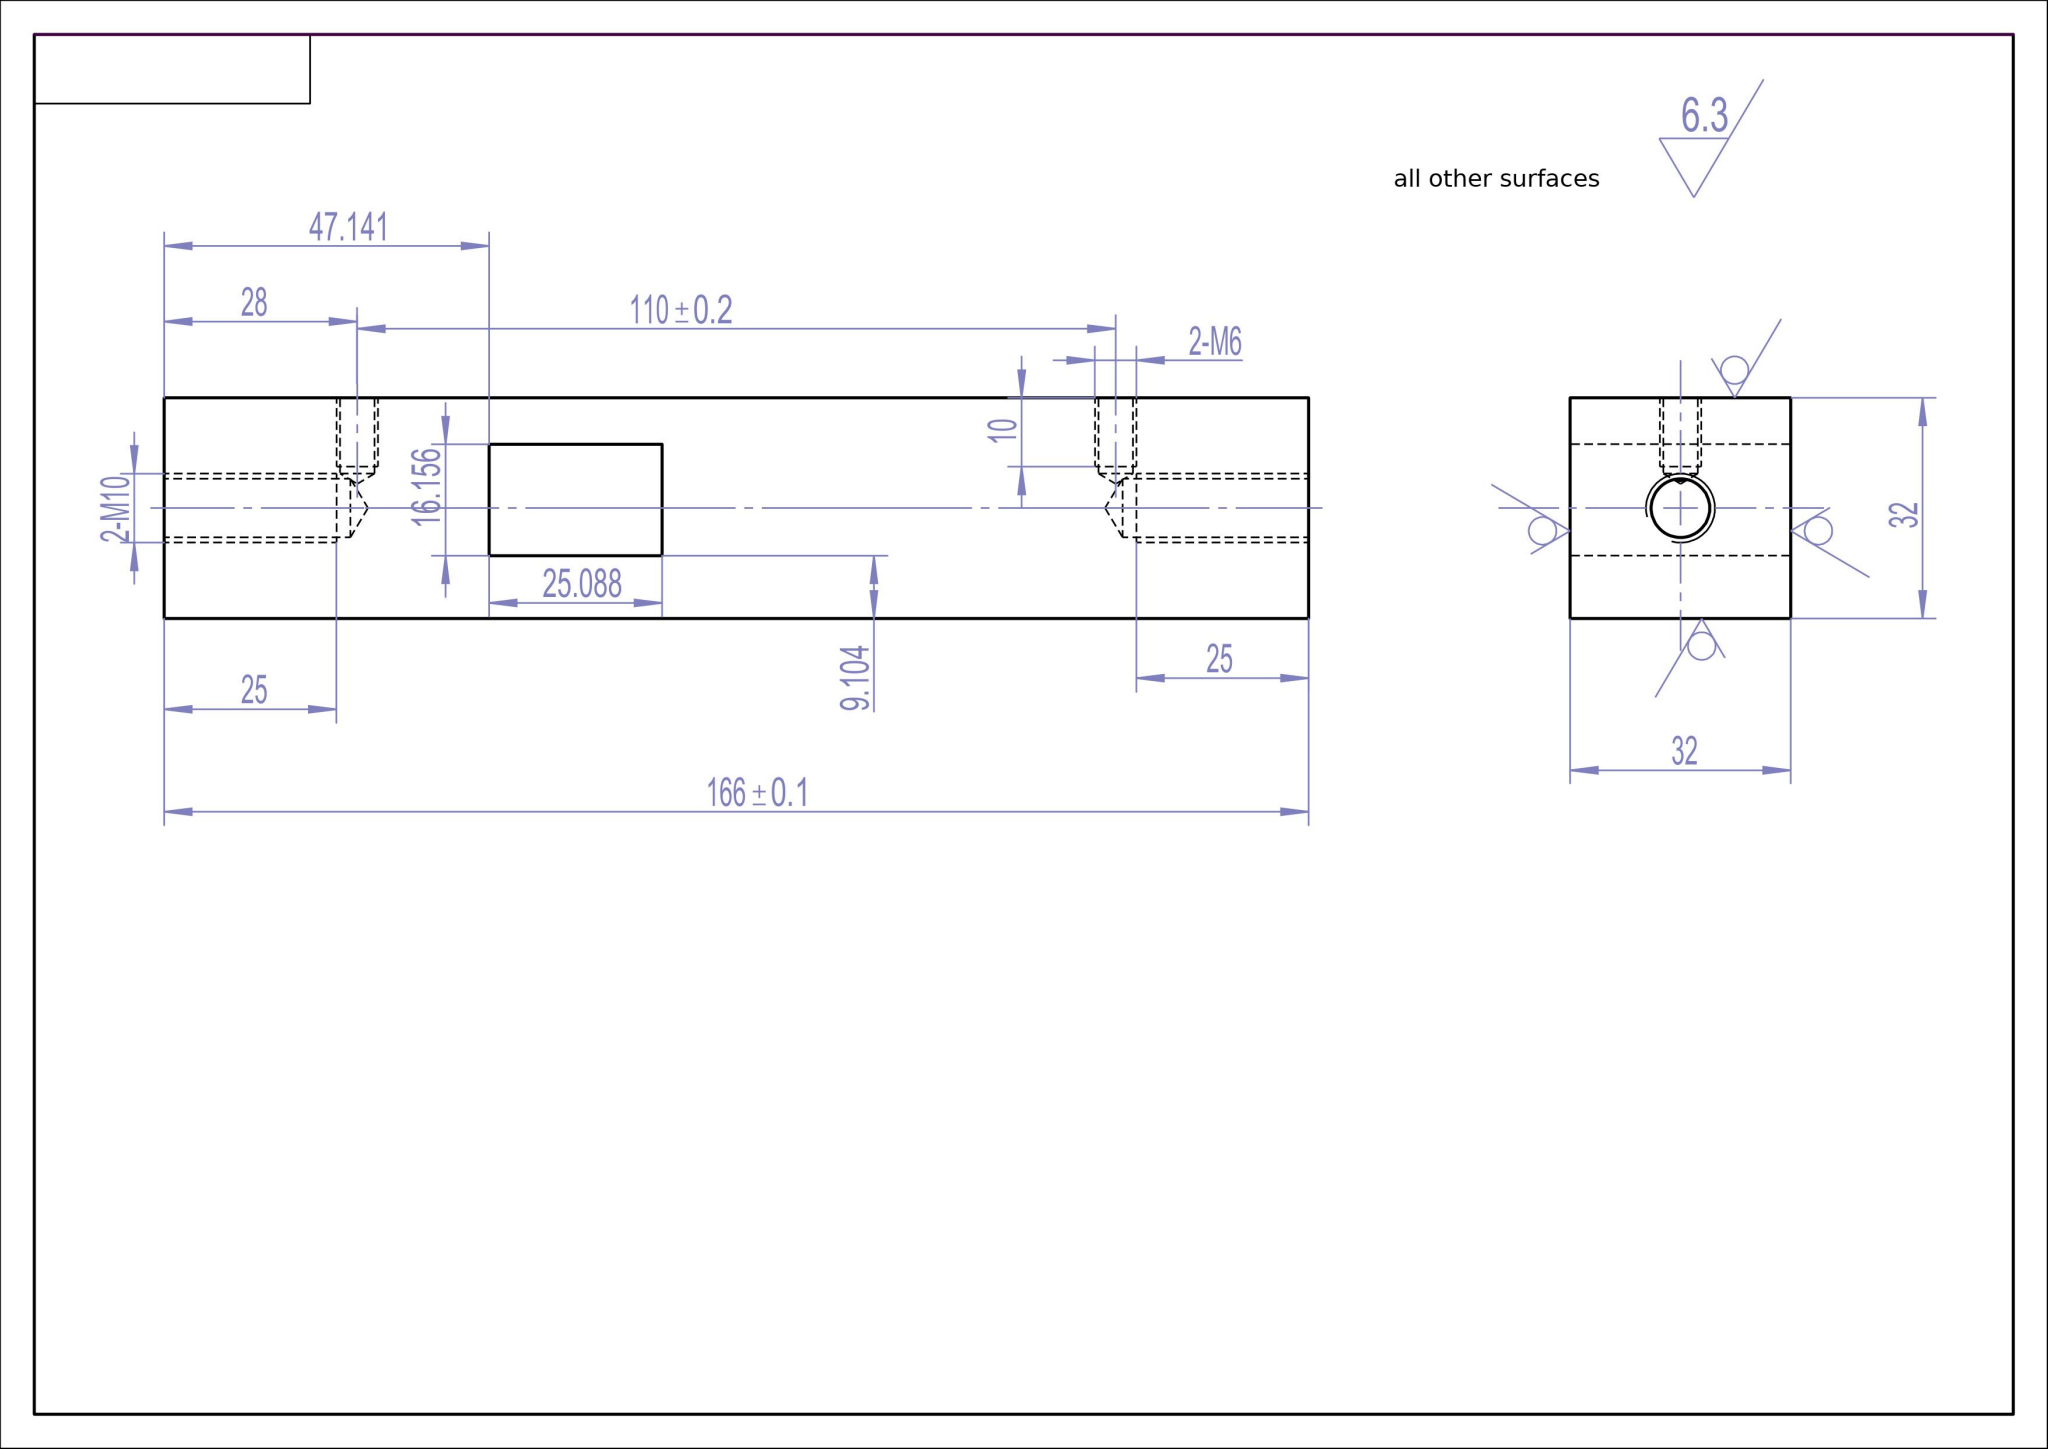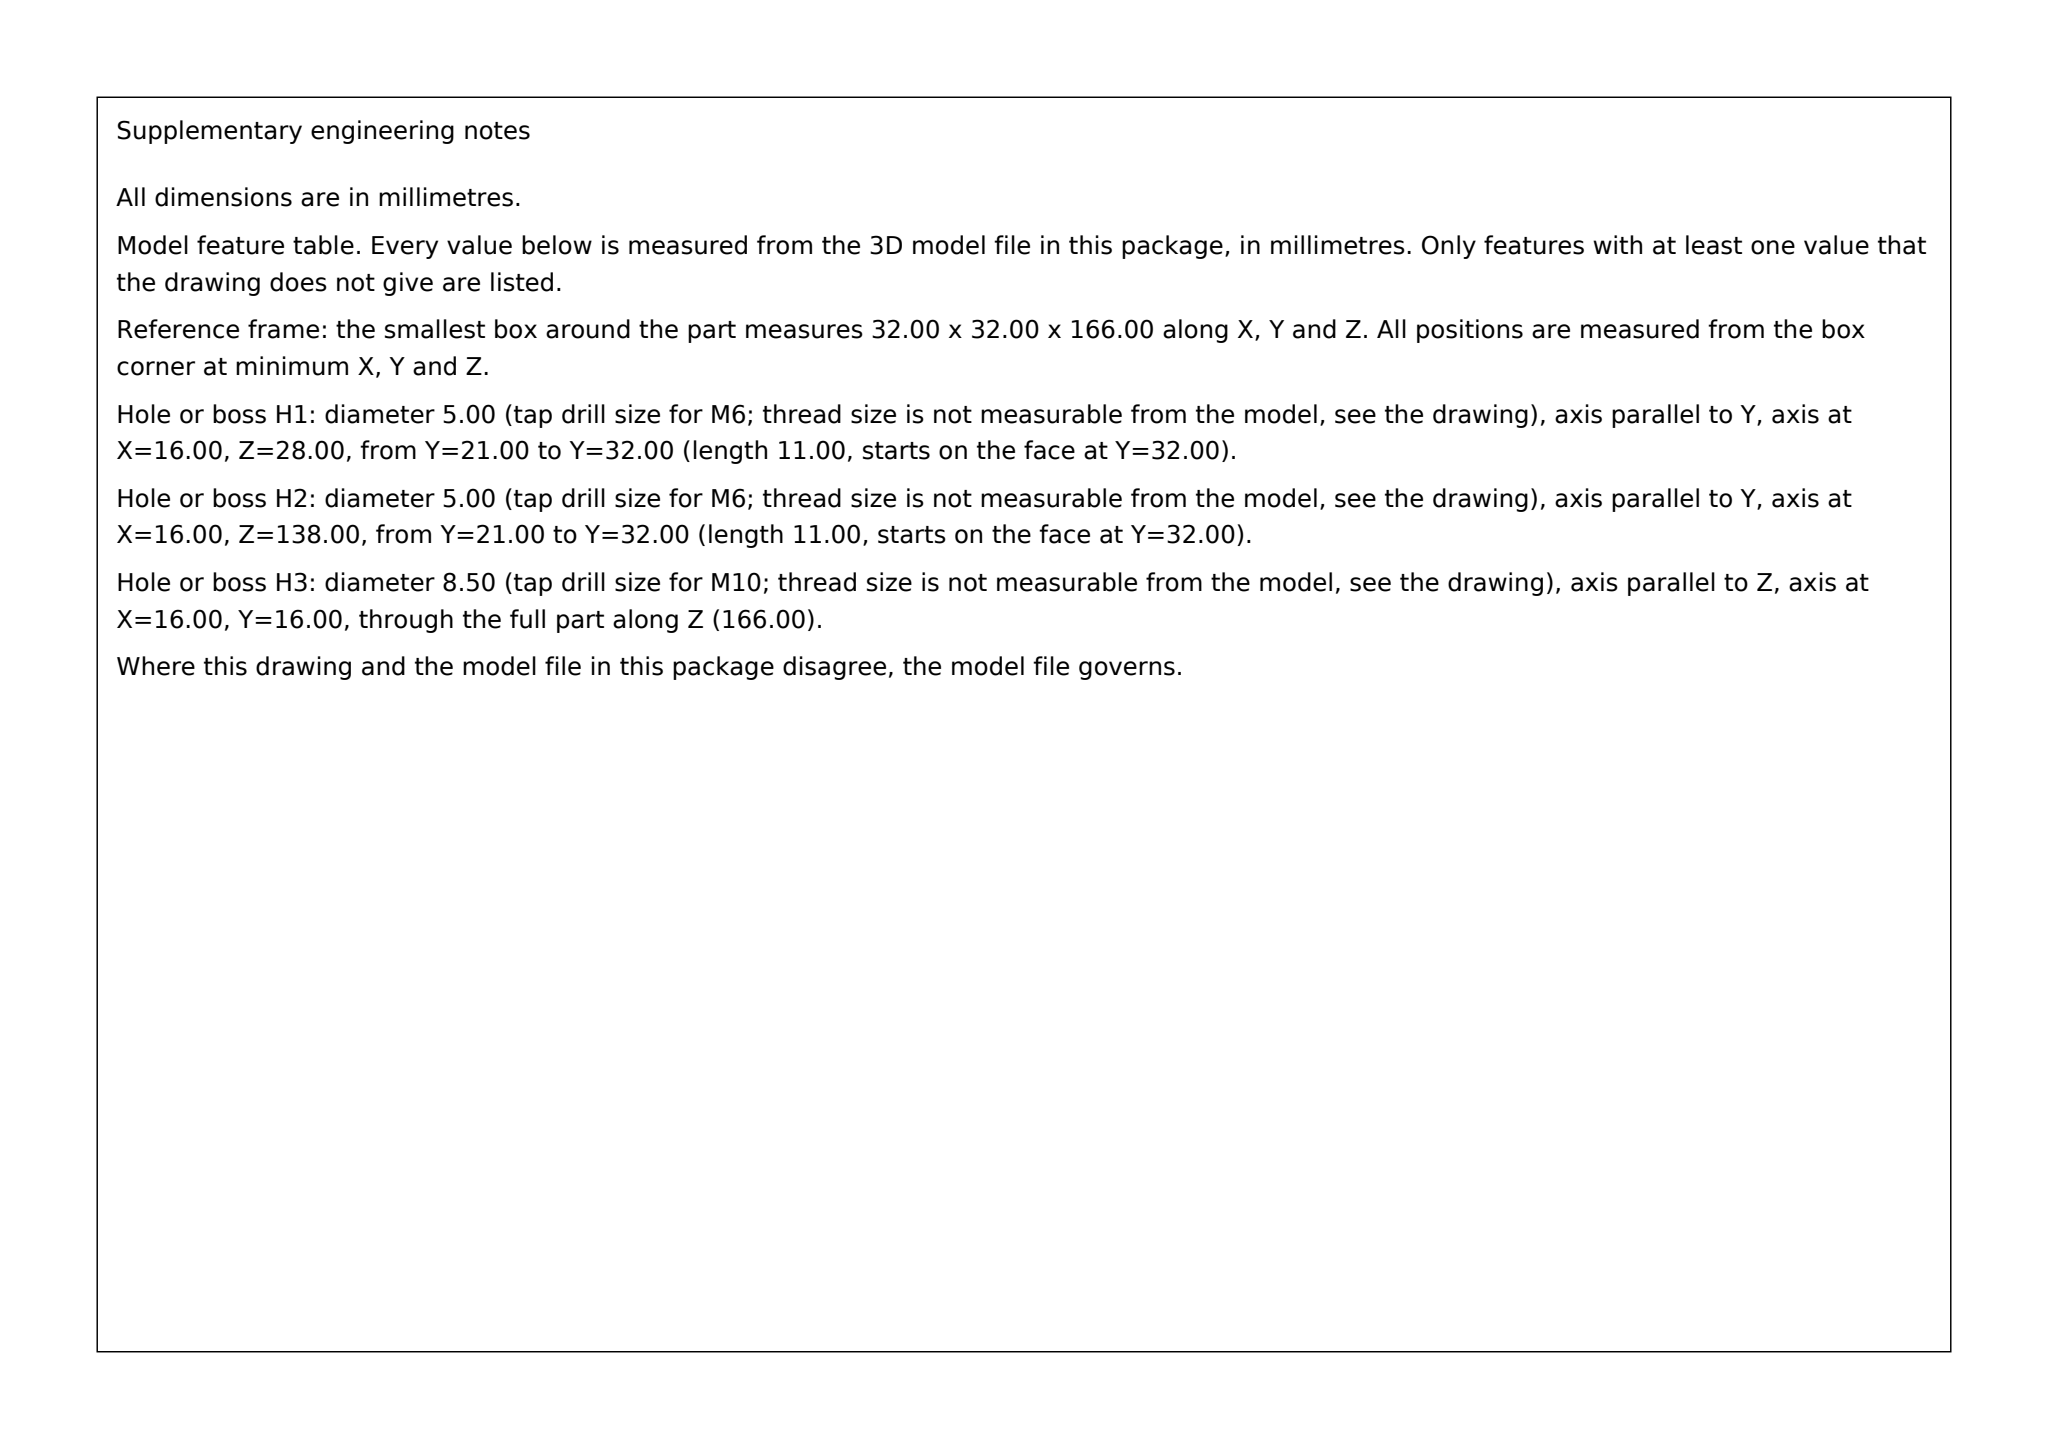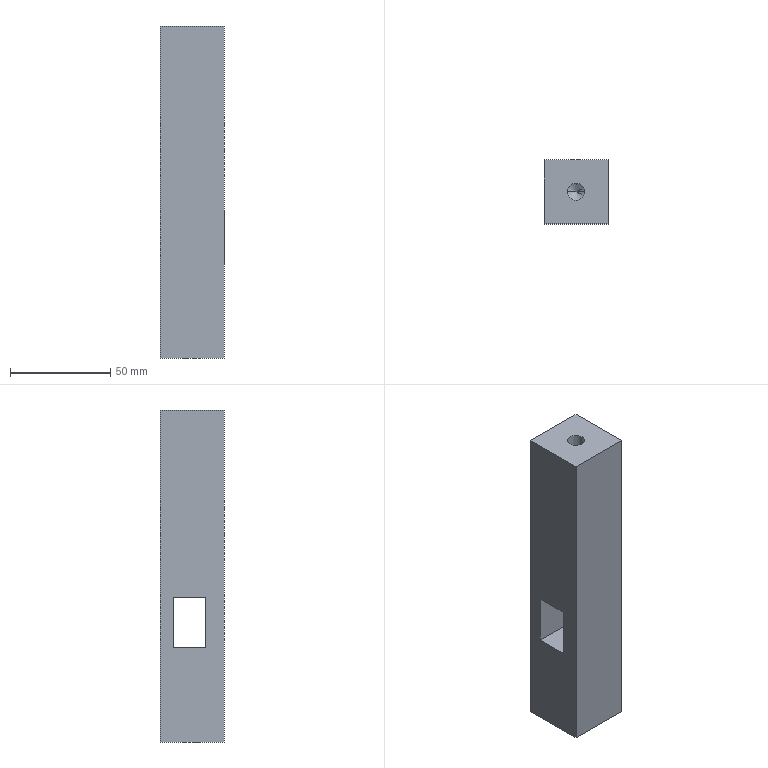Part | SolidWorks | mm | 1 solid | 26 faces | box 32 x 32 x 166 mm | volume 153401 mm3 | plane 10 | cylinder 8 | cone 8 | commonest cylinder face diameters 5 x4 8.5 x4
build123d program:
from build123d import *

# Parameters (mm, degrees)
SKETCH1_W           = 32
SKETCH1_H           = 32
BOSS_EXTRUDE1_DEPTH = 83
SKETCH6_W           = 25.088
SKETCH6_H           = 16.156
CUT_EXTRUDE1_DEPTH  = 77


with BuildPart() as part:
    # Sketch1 → Boss-Extrude1 (new, symmetric)
    with BuildSketch(Plane.XY):
        with Locations((-36.259, 1.485)):
            Rectangle(SKETCH1_W, SKETCH1_H)
    extrude(amount=BOSS_EXTRUDE1_DEPTH, both=True)

    # Sketch3 → M10 Tapped Hole1 (revolve, cut)
    with BuildSketch(Plane(origin=(-36.259, 1.485, 83), x_dir=(0, -1, 0), z_dir=(1, 0, 0))):
        Polygon((0, 0), (0, 29.554), (4.25, 27), (4.25, 0), align=None)
    m10_tapped_hole1 = revolve(axis=Axis((-36.259, 1.485, 89.35), (0, 0, -1)), mode=Mode.SUBTRACT)

    # Sketch5 → M6 Tapped Hole1 (revolve, cut)
    with BuildSketch(Plane(origin=(-36.259, 17.485, -55), x_dir=(0, 0, 1), z_dir=(1, 0, 0))):
        Polygon((0, 0), (0, 12.502), (2.5, 11), (2.5, 0), align=None)
    m6_tapped_hole1 = revolve(axis=Axis((-36.259, 23.835, -55), (0, -1, 0)), mode=Mode.SUBTRACT)

    # Mirror1: M10 Tapped Hole1, M6 Tapped Hole1 across plane
    add(m10_tapped_hole1.mirror(Plane.XY), mode=Mode.SUBTRACT)
    add(m6_tapped_hole1.mirror(Plane.XY), mode=Mode.SUBTRACT)

    # Sketch6 → Cut-Extrude1 (cut)
    with BuildSketch(Plane.ZY.offset(52.259)):
        with Locations((-23.315, 2.667)):
            Rectangle(SKETCH6_W, SKETCH6_H)
    extrude(amount=-CUT_EXTRUDE1_DEPTH, mode=Mode.SUBTRACT)


solid = part.part
STEP:
#1=CARTESIAN_POINT('',(-36.259,6.485,52.5));
#2=VERTEX_POINT('',#1);
#3=CARTESIAN_POINT('',(-36.259,6.485,57.5));
#4=VERTEX_POINT('',#3);
#5=CARTESIAN_POINT('',(-36.259,6.485,55.));
#6=DIRECTION('',(0.,1.,0.));
#7=DIRECTION('',(0.,0.,1.));
#8=AXIS2_PLACEMENT_3D('',#5,#6,#7);
#9=CIRCLE('',#8,2.5);
#10=EDGE_CURVE('',#2,#4,#9,.T.);
#11=ORIENTED_EDGE('',*,*,#10,.F.);
#12=CARTESIAN_POINT('',(-36.259,17.485,52.5));
#13=VERTEX_POINT('',#12);
#14=CARTESIAN_POINT('',(-36.259,17.485,52.5));
#15=DIRECTION('',(0.,1.,0.));
#16=VECTOR('',#15,1000.);
#17=LINE('',#14,#16);
#18=EDGE_CURVE('',#2,#13,#17,.T.);
#19=ORIENTED_EDGE('',*,*,#18,.T.);
#20=CARTESIAN_POINT('',(-36.259,17.485,57.5));
#21=VERTEX_POINT('',#20);
#22=CARTESIAN_POINT('',(-36.259,17.485,55.));
#23=DIRECTION('',(0.,1.,0.));
#24=DIRECTION('',(0.,0.,1.));
#25=AXIS2_PLACEMENT_3D('',#22,#23,#24);
#26=CIRCLE('',#25,2.5);
#27=EDGE_CURVE('',#13,#21,#26,.T.);
#28=ORIENTED_EDGE('',*,*,#27,.T.);
#29=CARTESIAN_POINT('',(-36.259,17.485,57.5));
#30=DIRECTION('',(0.,1.,0.));
#31=VECTOR('',#30,1000.);
#32=LINE('',#29,#31);
#33=EDGE_CURVE('',#4,#21,#32,.T.);
#34=ORIENTED_EDGE('',*,*,#33,.F.);
#35=EDGE_LOOP('',(#11,#19,#28,#34));
#36=FACE_OUTER_BOUND('',#35,.T.);
#37=CARTESIAN_POINT('',(-36.259,17.485,55.));
#38=DIRECTION('',(0.,1.,0.));
#39=DIRECTION('',(0.,0.,1.));
#40=AXIS2_PLACEMENT_3D('',#37,#38,#39);
#41=CYLINDRICAL_SURFACE('',#40,2.5);
#42=ADVANCED_FACE('',(#36),#41,.F.);
#43=CARTESIAN_POINT('',(-36.259,4.983,55.));
#44=VERTEX_POINT('',#43);
#45=CARTESIAN_POINT('',(-36.259,5.498,55.858));
#46=VERTEX_POINT('',#45);
#47=CARTESIAN_POINT('',(-36.259,6.485,57.5));
#48=DIRECTION('',(0.,0.515,0.8572));
#49=VECTOR('',#48,1000.);
#50=LINE('',#47,#49);
#51=EDGE_CURVE('',#44,#46,#50,.T.);
#52=ORIENTED_EDGE('',*,*,#51,.F.);
#53=CARTESIAN_POINT('',(-36.259,6.485,52.5));
#54=DIRECTION('',(0.,0.515,-0.8572));
#55=VECTOR('',#54,1000.);
#56=LINE('',#53,#55);
#57=EDGE_CURVE('',#44,#2,#56,.T.);
#58=ORIENTED_EDGE('',*,*,#57,.T.);
#59=ORIENTED_EDGE('',*,*,#10,.T.);
#60=CARTESIAN_POINT('',(-36.259,5.735,56.252));
#61=VERTEX_POINT('',#60);
#62=CARTESIAN_POINT('',(-36.259,6.485,57.5));
#63=DIRECTION('',(0.,0.515,0.8572));
#64=VECTOR('',#63,1000.);
#65=LINE('',#62,#64);
#66=EDGE_CURVE('',#61,#4,#65,.T.);
#67=ORIENTED_EDGE('',*,*,#66,.F.);
#68=CARTESIAN_POINT('',(-36.879,5.69,56.));
#69=VERTEX_POINT('',#68);
#70=CARTESIAN_POINT('',(-36.879,5.69,56.));
#71=CARTESIAN_POINT('',(-36.795,5.702,56.076));
#72=CARTESIAN_POINT('',(-36.698,5.714,56.14));
#73=CARTESIAN_POINT('',(-36.488,5.73,56.228));
#74=CARTESIAN_POINT('',(-36.373,5.735,56.252));
#75=CARTESIAN_POINT('',(-36.259,5.735,56.252));
#76=B_SPLINE_CURVE_WITH_KNOTS('',3,(#70,#71,#72,#73,#74,#75),.UNSPECIFIED.,.F.,.F.,(4,2,4),(0.0002047,0.0005456,0.0008865),.UNSPECIFIED.);
#77=EDGE_CURVE('',#69,#61,#76,.T.);
#78=ORIENTED_EDGE('',*,*,#77,.F.);
#79=CARTESIAN_POINT('',(-36.259,5.498,55.858));
#80=CARTESIAN_POINT('',(-36.372,5.498,55.858));
#81=CARTESIAN_POINT('',(-36.483,5.524,55.876));
#82=CARTESIAN_POINT('',(-36.688,5.595,55.929));
#83=CARTESIAN_POINT('',(-36.785,5.641,55.963));
#84=CARTESIAN_POINT('',(-36.879,5.69,56.));
#85=B_SPLINE_CURVE_WITH_KNOTS('',3,(#79,#80,#81,#82,#83,#84),.UNSPECIFIED.,.F.,.F.,(4,2,4),(0.0006719,0.001008,0.001345),.UNSPECIFIED.);
#86=EDGE_CURVE('',#46,#69,#85,.T.);
#87=ORIENTED_EDGE('',*,*,#86,.F.);
#88=EDGE_LOOP('',(#52,#58,#59,#67,#78,#87));
#89=FACE_OUTER_BOUND('',#88,.T.);
#90=CARTESIAN_POINT('',(-36.259,6.485,55.));
#91=DIRECTION('',(0.,1.,0.));
#92=DIRECTION('',(0.,0.,1.));
#93=AXIS2_PLACEMENT_3D('',#90,#91,#92);
#94=CONICAL_SURFACE('',#93,2.5,1.03);
#95=ADVANCED_FACE('',(#89),#94,.F.);
#96=CARTESIAN_POINT('',(-32.009,1.485,-56.));
#97=VERTEX_POINT('',#96);
#98=CARTESIAN_POINT('',(-40.509,1.485,-56.));
#99=VERTEX_POINT('',#98);
#100=CARTESIAN_POINT('',(-36.259,1.485,-56.));
#101=DIRECTION('',(0.,0.,-1.));
#102=DIRECTION('',(-1.,0.,0.));
#103=AXIS2_PLACEMENT_3D('',#100,#101,#102);
#104=CIRCLE('',#103,4.25);
#105=EDGE_CURVE('',#97,#99,#104,.T.);
#106=ORIENTED_EDGE('',*,*,#105,.F.);
#107=CARTESIAN_POINT('',(-32.009,1.485,-83.));
#108=VERTEX_POINT('',#107);
#109=CARTESIAN_POINT('',(-32.009,1.485,-83.));
#110=DIRECTION('',(0.,0.,-1.));
#111=VECTOR('',#110,1000.);
#112=LINE('',#109,#111);
#113=EDGE_CURVE('',#97,#108,#112,.T.);
#114=ORIENTED_EDGE('',*,*,#113,.T.);
#115=CARTESIAN_POINT('',(-40.509,1.485,-83.));
#116=VERTEX_POINT('',#115);
#117=CARTESIAN_POINT('',(-36.259,1.485,-83.));
#118=DIRECTION('',(0.,0.,-1.));
#119=DIRECTION('',(-1.,0.,0.));
#120=AXIS2_PLACEMENT_3D('',#117,#118,#119);
#121=CIRCLE('',#120,4.25);
#122=EDGE_CURVE('',#108,#116,#121,.T.);
#123=ORIENTED_EDGE('',*,*,#122,.T.);
#124=CARTESIAN_POINT('',(-40.509,1.485,-83.));
#125=DIRECTION('',(0.,0.,-1.));
#126=VECTOR('',#125,1000.);
#127=LINE('',#124,#126);
#128=EDGE_CURVE('',#99,#116,#127,.T.);
#129=ORIENTED_EDGE('',*,*,#128,.F.);
#130=EDGE_LOOP('',(#106,#114,#123,#129));
#131=FACE_OUTER_BOUND('',#130,.T.);
#132=CARTESIAN_POINT('',(-36.259,1.485,-83.));
#133=DIRECTION('',(0.,0.,-1.));
#134=DIRECTION('',(-1.,0.,0.));
#135=AXIS2_PLACEMENT_3D('',#132,#133,#134);
#136=CYLINDRICAL_SURFACE('',#135,4.25);
#137=ADVANCED_FACE('',(#131),#136,.F.);
#138=CARTESIAN_POINT('',(-36.259,1.485,-53.446));
#139=VERTEX_POINT('',#138);
#140=CARTESIAN_POINT('',(-40.509,1.485,-56.));
#141=DIRECTION('',(-0.8572,0.,-0.515));
#142=VECTOR('',#141,1000.);
#143=LINE('',#140,#142);
#144=EDGE_CURVE('',#139,#99,#143,.T.);
#145=ORIENTED_EDGE('',*,*,#144,.F.);
#146=CARTESIAN_POINT('',(-32.009,1.485,-56.));
#147=DIRECTION('',(0.8572,0.,-0.515));
#148=VECTOR('',#147,1000.);
#149=LINE('',#146,#148);
#150=EDGE_CURVE('',#139,#97,#149,.T.);
#151=ORIENTED_EDGE('',*,*,#150,.T.);
#152=ORIENTED_EDGE('',*,*,#105,.T.);
#153=EDGE_LOOP('',(#145,#151,#152));
#154=FACE_OUTER_BOUND('',#153,.T.);
#155=CARTESIAN_POINT('',(-36.259,1.485,-56.));
#156=DIRECTION('',(0.,0.,-1.));
#157=DIRECTION('',(-1.,0.,0.));
#158=AXIS2_PLACEMENT_3D('',#155,#156,#157);
#159=CONICAL_SURFACE('',#158,4.25,1.03);
#160=ADVANCED_FACE('',(#154),#159,.F.);
#161=CARTESIAN_POINT('',(-36.259,6.485,-57.5));
#162=VERTEX_POINT('',#161);
#163=CARTESIAN_POINT('',(-36.259,6.485,-52.5));
#164=VERTEX_POINT('',#163);
#165=CARTESIAN_POINT('',(-36.259,6.485,-55.));
#166=DIRECTION('',(0.,1.,0.));
#167=DIRECTION('',(0.,0.,1.));
#168=AXIS2_PLACEMENT_3D('',#165,#166,#167);
#169=CIRCLE('',#168,2.5);
#170=EDGE_CURVE('',#162,#164,#169,.T.);
#171=ORIENTED_EDGE('',*,*,#170,.F.);
#172=CARTESIAN_POINT('',(-36.259,17.485,-57.5));
#173=VERTEX_POINT('',#172);
#174=CARTESIAN_POINT('',(-36.259,17.485,-57.5));
#175=DIRECTION('',(0.,1.,0.));
#176=VECTOR('',#175,1000.);
#177=LINE('',#174,#176);
#178=EDGE_CURVE('',#162,#173,#177,.T.);
#179=ORIENTED_EDGE('',*,*,#178,.T.);
#180=CARTESIAN_POINT('',(-36.259,17.485,-52.5));
#181=VERTEX_POINT('',#180);
#182=CARTESIAN_POINT('',(-36.259,17.485,-55.));
#183=DIRECTION('',(0.,1.,0.));
#184=DIRECTION('',(0.,0.,1.));
#185=AXIS2_PLACEMENT_3D('',#182,#183,#184);
#186=CIRCLE('',#185,2.5);
#187=EDGE_CURVE('',#173,#181,#186,.T.);
#188=ORIENTED_EDGE('',*,*,#187,.T.);
#189=CARTESIAN_POINT('',(-36.259,17.485,-52.5));
#190=DIRECTION('',(0.,1.,0.));
#191=VECTOR('',#190,1000.);
#192=LINE('',#189,#191);
#193=EDGE_CURVE('',#164,#181,#192,.T.);
#194=ORIENTED_EDGE('',*,*,#193,.F.);
#195=EDGE_LOOP('',(#171,#179,#188,#194));
#196=FACE_OUTER_BOUND('',#195,.T.);
#197=CARTESIAN_POINT('',(-36.259,17.485,-55.));
#198=DIRECTION('',(0.,1.,0.));
#199=DIRECTION('',(0.,0.,1.));
#200=AXIS2_PLACEMENT_3D('',#197,#198,#199);
#201=CYLINDRICAL_SURFACE('',#200,2.5);
#202=ADVANCED_FACE('',(#196),#201,.F.);
#203=CARTESIAN_POINT('',(-36.259,4.983,-55.));
#204=VERTEX_POINT('',#203);
#205=CARTESIAN_POINT('',(-36.259,6.485,-52.5));
#206=DIRECTION('',(0.,0.515,0.8572));
#207=VECTOR('',#206,1000.);
#208=LINE('',#205,#207);
#209=EDGE_CURVE('',#204,#164,#208,.T.);
#210=ORIENTED_EDGE('',*,*,#209,.F.);
#211=CARTESIAN_POINT('',(-36.259,5.498,-55.858));
#212=VERTEX_POINT('',#211);
#213=CARTESIAN_POINT('',(-36.259,6.485,-57.5));
#214=DIRECTION('',(0.,0.515,-0.8572));
#215=VECTOR('',#214,1000.);
#216=LINE('',#213,#215);
#217=EDGE_CURVE('',#204,#212,#216,.T.);
#218=ORIENTED_EDGE('',*,*,#217,.T.);
#219=CARTESIAN_POINT('',(-36.879,5.69,-56.));
#220=VERTEX_POINT('',#219);
#221=CARTESIAN_POINT('',(-36.259,5.498,-55.858));
#222=CARTESIAN_POINT('',(-36.372,5.498,-55.858));
#223=CARTESIAN_POINT('',(-36.483,5.524,-55.876));
#224=CARTESIAN_POINT('',(-36.688,5.595,-55.929));
#225=CARTESIAN_POINT('',(-36.785,5.641,-55.963));
#226=CARTESIAN_POINT('',(-36.879,5.69,-56.));
#227=B_SPLINE_CURVE_WITH_KNOTS('',3,(#221,#222,#223,#224,#225,#226),.UNSPECIFIED.,.F.,.F.,(4,2,4),(0.0006719,0.001008,0.001345),.UNSPECIFIED.);
#228=EDGE_CURVE('',#212,#220,#227,.T.);
#229=ORIENTED_EDGE('',*,*,#228,.T.);
#230=CARTESIAN_POINT('',(-36.259,5.735,-56.252));
#231=VERTEX_POINT('',#230);
#232=CARTESIAN_POINT('',(-36.879,5.69,-56.));
#233=CARTESIAN_POINT('',(-36.795,5.702,-56.076));
#234=CARTESIAN_POINT('',(-36.698,5.714,-56.14));
#235=CARTESIAN_POINT('',(-36.488,5.73,-56.228));
#236=CARTESIAN_POINT('',(-36.373,5.735,-56.252));
#237=CARTESIAN_POINT('',(-36.259,5.735,-56.252));
#238=B_SPLINE_CURVE_WITH_KNOTS('',3,(#232,#233,#234,#235,#236,#237),.UNSPECIFIED.,.F.,.F.,(4,2,4),(0.0002047,0.0005456,0.0008865),.UNSPECIFIED.);
#239=EDGE_CURVE('',#220,#231,#238,.T.);
#240=ORIENTED_EDGE('',*,*,#239,.T.);
#241=CARTESIAN_POINT('',(-36.259,6.485,-57.5));
#242=DIRECTION('',(0.,0.515,-0.8572));
#243=VECTOR('',#242,1000.);
#244=LINE('',#241,#243);
#245=EDGE_CURVE('',#231,#162,#244,.T.);
#246=ORIENTED_EDGE('',*,*,#245,.T.);
#247=ORIENTED_EDGE('',*,*,#170,.T.);
#248=EDGE_LOOP('',(#210,#218,#229,#240,#246,#247));
#249=FACE_OUTER_BOUND('',#248,.T.);
#250=CARTESIAN_POINT('',(-36.259,6.485,-55.));
#251=DIRECTION('',(0.,1.,0.));
#252=DIRECTION('',(0.,0.,1.));
#253=AXIS2_PLACEMENT_3D('',#250,#251,#252);
#254=CONICAL_SURFACE('',#253,2.5,1.03);
#255=ADVANCED_FACE('',(#249),#254,.F.);
#256=CARTESIAN_POINT('',(-40.509,1.485,56.));
#257=VERTEX_POINT('',#256);
#258=CARTESIAN_POINT('',(-32.009,1.485,56.));
#259=VERTEX_POINT('',#258);
#260=CARTESIAN_POINT('',(-36.259,1.485,56.));
#261=DIRECTION('',(0.,0.,1.));
#262=DIRECTION('',(1.,0.,0.));
#263=AXIS2_PLACEMENT_3D('',#260,#261,#262);
#264=CIRCLE('',#263,4.25);
#265=EDGE_CURVE('',#257,#259,#264,.T.);
#266=ORIENTED_EDGE('',*,*,#265,.F.);
#267=CARTESIAN_POINT('',(-40.509,1.485,83.));
#268=VERTEX_POINT('',#267);
#269=CARTESIAN_POINT('',(-40.509,1.485,83.));
#270=DIRECTION('',(0.,0.,1.));
#271=VECTOR('',#270,1000.);
#272=LINE('',#269,#271);
#273=EDGE_CURVE('',#257,#268,#272,.T.);
#274=ORIENTED_EDGE('',*,*,#273,.T.);
#275=CARTESIAN_POINT('',(-32.009,1.485,83.));
#276=VERTEX_POINT('',#275);
#277=CARTESIAN_POINT('',(-36.259,1.485,83.));
#278=DIRECTION('',(0.,0.,1.));
#279=DIRECTION('',(1.,0.,0.));
#280=AXIS2_PLACEMENT_3D('',#277,#278,#279);
#281=CIRCLE('',#280,4.25);
#282=EDGE_CURVE('',#268,#276,#281,.T.);
#283=ORIENTED_EDGE('',*,*,#282,.T.);
#284=CARTESIAN_POINT('',(-32.009,1.485,83.));
#285=DIRECTION('',(0.,0.,1.));
#286=VECTOR('',#285,1000.);
#287=LINE('',#284,#286);
#288=EDGE_CURVE('',#259,#276,#287,.T.);
#289=ORIENTED_EDGE('',*,*,#288,.F.);
#290=EDGE_LOOP('',(#266,#274,#283,#289));
#291=FACE_OUTER_BOUND('',#290,.T.);
#292=CARTESIAN_POINT('',(-36.259,1.485,83.));
#293=DIRECTION('',(0.,0.,1.));
#294=DIRECTION('',(1.,0.,0.));
#295=AXIS2_PLACEMENT_3D('',#292,#293,#294);
#296=CYLINDRICAL_SURFACE('',#295,4.25);
#297=ADVANCED_FACE('',(#291),#296,.F.);
#298=CARTESIAN_POINT('',(-36.259,1.485,53.446));
#299=VERTEX_POINT('',#298);
#300=CARTESIAN_POINT('',(-32.009,1.485,56.));
#301=DIRECTION('',(0.8572,0.,0.515));
#302=VECTOR('',#301,1000.);
#303=LINE('',#300,#302);
#304=EDGE_CURVE('',#299,#259,#303,.T.);
#305=ORIENTED_EDGE('',*,*,#304,.F.);
#306=CARTESIAN_POINT('',(-40.509,1.485,56.));
#307=DIRECTION('',(-0.8572,0.,0.515));
#308=VECTOR('',#307,1000.);
#309=LINE('',#306,#308);
#310=EDGE_CURVE('',#299,#257,#309,.T.);
#311=ORIENTED_EDGE('',*,*,#310,.T.);
#312=ORIENTED_EDGE('',*,*,#265,.T.);
#313=EDGE_LOOP('',(#305,#311,#312));
#314=FACE_OUTER_BOUND('',#313,.T.);
#315=CARTESIAN_POINT('',(-36.259,1.485,56.));
#316=DIRECTION('',(0.,0.,1.));
#317=DIRECTION('',(1.,0.,0.));
#318=AXIS2_PLACEMENT_3D('',#315,#316,#317);
#319=CONICAL_SURFACE('',#318,4.25,1.03);
#320=ADVANCED_FACE('',(#314),#319,.F.);
#321=CARTESIAN_POINT('',(-52.259,-5.411,-35.859));
#322=VERTEX_POINT('',#321);
#323=CARTESIAN_POINT('',(-52.259,-5.411,-10.771));
#324=VERTEX_POINT('',#323);
#325=CARTESIAN_POINT('',(-52.259,-5.411,-35.859));
#326=DIRECTION('',(0.,0.,1.));
#327=VECTOR('',#326,1000.);
#328=LINE('',#325,#327);
#329=EDGE_CURVE('',#322,#324,#328,.T.);
#330=ORIENTED_EDGE('',*,*,#329,.F.);
#331=CARTESIAN_POINT('',(-52.259,10.746,-35.859));
#332=VERTEX_POINT('',#331);
#333=CARTESIAN_POINT('',(-52.259,10.746,-35.859));
#334=DIRECTION('',(0.,-1.,0.));
#335=VECTOR('',#334,1000.);
#336=LINE('',#333,#335);
#337=EDGE_CURVE('',#332,#322,#336,.T.);
#338=ORIENTED_EDGE('',*,*,#337,.F.);
#339=CARTESIAN_POINT('',(-52.259,10.746,-10.771));
#340=VERTEX_POINT('',#339);
#341=CARTESIAN_POINT('',(-52.259,10.746,-35.859));
#342=DIRECTION('',(0.,0.,-1.));
#343=VECTOR('',#342,1000.);
#344=LINE('',#341,#343);
#345=EDGE_CURVE('',#340,#332,#344,.T.);
#346=ORIENTED_EDGE('',*,*,#345,.F.);
#347=CARTESIAN_POINT('',(-52.259,10.746,-10.771));
#348=DIRECTION('',(0.,1.,0.));
#349=VECTOR('',#348,1000.);
#350=LINE('',#347,#349);
#351=EDGE_CURVE('',#324,#340,#350,.T.);
#352=ORIENTED_EDGE('',*,*,#351,.F.);
#353=EDGE_LOOP('',(#330,#338,#346,#352));
#354=FACE_BOUND('',#353,.T.);
#355=CARTESIAN_POINT('',(-52.259,17.485,-83.));
#356=VERTEX_POINT('',#355);
#357=CARTESIAN_POINT('',(-52.259,-14.515,-83.));
#358=VERTEX_POINT('',#357);
#359=CARTESIAN_POINT('',(-52.259,17.485,-83.));
#360=DIRECTION('',(0.,-1.,0.));
#361=VECTOR('',#360,1000.);
#362=LINE('',#359,#361);
#363=EDGE_CURVE('',#356,#358,#362,.T.);
#364=ORIENTED_EDGE('',*,*,#363,.T.);
#365=CARTESIAN_POINT('',(-52.259,-14.515,83.));
#366=VERTEX_POINT('',#365);
#367=CARTESIAN_POINT('',(-52.259,-14.515,83.));
#368=DIRECTION('',(0.,0.,-1.));
#369=VECTOR('',#368,1000.);
#370=LINE('',#367,#369);
#371=EDGE_CURVE('',#366,#358,#370,.T.);
#372=ORIENTED_EDGE('',*,*,#371,.F.);
#373=CARTESIAN_POINT('',(-52.259,17.485,83.));
#374=VERTEX_POINT('',#373);
#375=CARTESIAN_POINT('',(-52.259,17.485,83.));
#376=DIRECTION('',(0.,-1.,0.));
#377=VECTOR('',#376,1000.);
#378=LINE('',#375,#377);
#379=EDGE_CURVE('',#374,#366,#378,.T.);
#380=ORIENTED_EDGE('',*,*,#379,.F.);
#381=CARTESIAN_POINT('',(-52.259,17.485,83.));
#382=DIRECTION('',(0.,0.,-1.));
#383=VECTOR('',#382,1000.);
#384=LINE('',#381,#383);
#385=EDGE_CURVE('',#374,#356,#384,.T.);
#386=ORIENTED_EDGE('',*,*,#385,.T.);
#387=EDGE_LOOP('',(#364,#372,#380,#386));
#388=FACE_OUTER_BOUND('',#387,.T.);
#389=CARTESIAN_POINT('',(-52.259,17.485,83.));
#390=DIRECTION('',(1.,0.,0.));
#391=DIRECTION('',(0.,0.,-1.));
#392=AXIS2_PLACEMENT_3D('',#389,#390,#391);
#393=PLANE('',#392);
#394=ADVANCED_FACE('',(#354,#388),#393,.F.);
#395=CARTESIAN_POINT('',(-20.259,-14.515,-83.));
#396=VERTEX_POINT('',#395);
#397=CARTESIAN_POINT('',(-52.259,-14.515,-83.));
#398=DIRECTION('',(1.,0.,0.));
#399=VECTOR('',#398,1000.);
#400=LINE('',#397,#399);
#401=EDGE_CURVE('',#358,#396,#400,.T.);
#402=ORIENTED_EDGE('',*,*,#401,.T.);
#403=CARTESIAN_POINT('',(-20.259,-14.515,83.));
#404=VERTEX_POINT('',#403);
#405=CARTESIAN_POINT('',(-20.259,-14.515,83.));
#406=DIRECTION('',(0.,0.,-1.));
#407=VECTOR('',#406,1000.);
#408=LINE('',#405,#407);
#409=EDGE_CURVE('',#404,#396,#408,.T.);
#410=ORIENTED_EDGE('',*,*,#409,.F.);
#411=CARTESIAN_POINT('',(-52.259,-14.515,83.));
#412=DIRECTION('',(1.,0.,0.));
#413=VECTOR('',#412,1000.);
#414=LINE('',#411,#413);
#415=EDGE_CURVE('',#366,#404,#414,.T.);
#416=ORIENTED_EDGE('',*,*,#415,.F.);
#417=ORIENTED_EDGE('',*,*,#371,.T.);
#418=EDGE_LOOP('',(#402,#410,#416,#417));
#419=FACE_OUTER_BOUND('',#418,.T.);
#420=CARTESIAN_POINT('',(-52.259,-14.515,83.));
#421=DIRECTION('',(0.,1.,0.));
#422=DIRECTION('',(0.,0.,1.));
#423=AXIS2_PLACEMENT_3D('',#420,#421,#422);
#424=PLANE('',#423);
#425=ADVANCED_FACE('',(#419),#424,.F.);
#426=CARTESIAN_POINT('',(-20.259,10.746,-10.771));
#427=VERTEX_POINT('',#426);
#428=CARTESIAN_POINT('',(-20.259,10.746,-35.859));
#429=VERTEX_POINT('',#428);
#430=CARTESIAN_POINT('',(-20.259,10.746,83.));
#431=DIRECTION('',(0.,0.,-1.));
#432=VECTOR('',#431,1000.);
#433=LINE('',#430,#432);
#434=EDGE_CURVE('',#427,#429,#433,.T.);
#435=ORIENTED_EDGE('',*,*,#434,.T.);
#436=CARTESIAN_POINT('',(-20.259,-5.411,-35.859));
#437=VERTEX_POINT('',#436);
#438=CARTESIAN_POINT('',(-20.259,17.485,-35.859));
#439=DIRECTION('',(0.,-1.,0.));
#440=VECTOR('',#439,1000.);
#441=LINE('',#438,#440);
#442=EDGE_CURVE('',#429,#437,#441,.T.);
#443=ORIENTED_EDGE('',*,*,#442,.T.);
#444=CARTESIAN_POINT('',(-20.259,-5.411,-10.771));
#445=VERTEX_POINT('',#444);
#446=CARTESIAN_POINT('',(-20.259,-5.411,83.));
#447=DIRECTION('',(0.,0.,1.));
#448=VECTOR('',#447,1000.);
#449=LINE('',#446,#448);
#450=EDGE_CURVE('',#437,#445,#449,.T.);
#451=ORIENTED_EDGE('',*,*,#450,.T.);
#452=CARTESIAN_POINT('',(-20.259,17.485,-10.771));
#453=DIRECTION('',(-0.,1.,0.));
#454=VECTOR('',#453,1000.);
#455=LINE('',#452,#454);
#456=EDGE_CURVE('',#445,#427,#455,.T.);
#457=ORIENTED_EDGE('',*,*,#456,.T.);
#458=EDGE_LOOP('',(#435,#443,#451,#457));
#459=FACE_BOUND('',#458,.T.);
#460=CARTESIAN_POINT('',(-20.259,17.485,-83.));
#461=VERTEX_POINT('',#460);
#462=CARTESIAN_POINT('',(-20.259,17.485,-83.));
#463=DIRECTION('',(-0.,1.,0.));
#464=VECTOR('',#463,1000.);
#465=LINE('',#462,#464);
#466=EDGE_CURVE('',#396,#461,#465,.T.);
#467=ORIENTED_EDGE('',*,*,#466,.T.);
#468=CARTESIAN_POINT('',(-20.259,17.485,83.));
#469=VERTEX_POINT('',#468);
#470=CARTESIAN_POINT('',(-20.259,17.485,83.));
#471=DIRECTION('',(0.,0.,-1.));
#472=VECTOR('',#471,1000.);
#473=LINE('',#470,#472);
#474=EDGE_CURVE('',#469,#461,#473,.T.);
#475=ORIENTED_EDGE('',*,*,#474,.F.);
#476=CARTESIAN_POINT('',(-20.259,17.485,83.));
#477=DIRECTION('',(-0.,1.,0.));
#478=VECTOR('',#477,1000.);
#479=LINE('',#476,#478);
#480=EDGE_CURVE('',#404,#469,#479,.T.);
#481=ORIENTED_EDGE('',*,*,#480,.F.);
#482=ORIENTED_EDGE('',*,*,#409,.T.);
#483=EDGE_LOOP('',(#467,#475,#481,#482));
#484=FACE_OUTER_BOUND('',#483,.T.);
#485=CARTESIAN_POINT('',(-20.259,17.485,83.));
#486=DIRECTION('',(-1.,-0.,0.));
#487=DIRECTION('',(0.,-1.,0.));
#488=AXIS2_PLACEMENT_3D('',#485,#486,#487);
#489=PLANE('',#488);
#490=ADVANCED_FACE('',(#459,#484),#489,.F.);
#491=CARTESIAN_POINT('',(-36.259,17.485,55.));
#492=DIRECTION('',(0.,1.,0.));
#493=DIRECTION('',(0.,0.,1.));
#494=AXIS2_PLACEMENT_3D('',#491,#492,#493);
#495=CIRCLE('',#494,2.5);
#496=EDGE_CURVE('',#21,#13,#495,.T.);
#497=ORIENTED_EDGE('',*,*,#496,.F.);
#498=ORIENTED_EDGE('',*,*,#27,.F.);
#499=EDGE_LOOP('',(#497,#498));
#500=FACE_BOUND('',#499,.T.);
#501=CARTESIAN_POINT('',(-36.259,17.485,-55.));
#502=DIRECTION('',(0.,1.,0.));
#503=DIRECTION('',(0.,0.,1.));
#504=AXIS2_PLACEMENT_3D('',#501,#502,#503);
#505=CIRCLE('',#504,2.5);
#506=EDGE_CURVE('',#181,#173,#505,.T.);
#507=ORIENTED_EDGE('',*,*,#506,.F.);
#508=ORIENTED_EDGE('',*,*,#187,.F.);
#509=EDGE_LOOP('',(#507,#508));
#510=FACE_BOUND('',#509,.T.);
#511=CARTESIAN_POINT('',(-52.259,17.485,-83.));
#512=DIRECTION('',(-1.,0.,0.));
#513=VECTOR('',#512,1000.);
#514=LINE('',#511,#513);
#515=EDGE_CURVE('',#461,#356,#514,.T.);
#516=ORIENTED_EDGE('',*,*,#515,.T.);
#517=ORIENTED_EDGE('',*,*,#385,.F.);
#518=CARTESIAN_POINT('',(-52.259,17.485,83.));
#519=DIRECTION('',(-1.,0.,0.));
#520=VECTOR('',#519,1000.);
#521=LINE('',#518,#520);
#522=EDGE_CURVE('',#469,#374,#521,.T.);
#523=ORIENTED_EDGE('',*,*,#522,.F.);
#524=ORIENTED_EDGE('',*,*,#474,.T.);
#525=EDGE_LOOP('',(#516,#517,#523,#524));
#526=FACE_OUTER_BOUND('',#525,.T.);
#527=CARTESIAN_POINT('',(-52.259,17.485,83.));
#528=DIRECTION('',(0.,-1.,0.));
#529=DIRECTION('',(0.,0.,-1.));
#530=AXIS2_PLACEMENT_3D('',#527,#528,#529);
#531=PLANE('',#530);
#532=ADVANCED_FACE('',(#500,#510,#526),#531,.F.);
#533=CARTESIAN_POINT('',(-36.259,1.485,83.));
#534=DIRECTION('',(0.,0.,1.));
#535=DIRECTION('',(1.,0.,0.));
#536=AXIS2_PLACEMENT_3D('',#533,#534,#535);
#537=CIRCLE('',#536,4.25);
#538=EDGE_CURVE('',#276,#268,#537,.T.);
#539=ORIENTED_EDGE('',*,*,#538,.F.);
#540=ORIENTED_EDGE('',*,*,#282,.F.);
#541=EDGE_LOOP('',(#539,#540));
#542=FACE_BOUND('',#541,.T.);
#543=ORIENTED_EDGE('',*,*,#379,.T.);
#544=ORIENTED_EDGE('',*,*,#415,.T.);
#545=ORIENTED_EDGE('',*,*,#480,.T.);
#546=ORIENTED_EDGE('',*,*,#522,.T.);
#547=EDGE_LOOP('',(#543,#544,#545,#546));
#548=FACE_OUTER_BOUND('',#547,.T.);
#549=CARTESIAN_POINT('',(0.,0.,83.));
#550=DIRECTION('',(0.,0.,1.));
#551=DIRECTION('',(1.,0.,0.));
#552=AXIS2_PLACEMENT_3D('',#549,#550,#551);
#553=PLANE('',#552);
#554=ADVANCED_FACE('',(#542,#548),#553,.T.);
#555=CARTESIAN_POINT('',(-36.259,1.485,-83.));
#556=DIRECTION('',(0.,0.,-1.));
#557=DIRECTION('',(-1.,0.,0.));
#558=AXIS2_PLACEMENT_3D('',#555,#556,#557);
#559=CIRCLE('',#558,4.25);
#560=EDGE_CURVE('',#116,#108,#559,.T.);
#561=ORIENTED_EDGE('',*,*,#560,.F.);
#562=ORIENTED_EDGE('',*,*,#122,.F.);
#563=EDGE_LOOP('',(#561,#562));
#564=FACE_BOUND('',#563,.T.);
#565=ORIENTED_EDGE('',*,*,#363,.F.);
#566=ORIENTED_EDGE('',*,*,#515,.F.);
#567=ORIENTED_EDGE('',*,*,#466,.F.);
#568=ORIENTED_EDGE('',*,*,#401,.F.);
#569=EDGE_LOOP('',(#565,#566,#567,#568));
#570=FACE_OUTER_BOUND('',#569,.T.);
#571=CARTESIAN_POINT('',(0.,0.,-83.));
#572=DIRECTION('',(0.,0.,1.));
#573=DIRECTION('',(1.,0.,0.));
#574=AXIS2_PLACEMENT_3D('',#571,#572,#573);
#575=PLANE('',#574);
#576=ADVANCED_FACE('',(#564,#570),#575,.F.);
#577=ORIENTED_EDGE('',*,*,#310,.F.);
#578=ORIENTED_EDGE('',*,*,#304,.T.);
#579=CARTESIAN_POINT('',(-35.64,5.69,56.));
#580=VERTEX_POINT('',#579);
#581=CARTESIAN_POINT('',(-36.259,1.485,56.));
#582=DIRECTION('',(0.,0.,1.));
#583=DIRECTION('',(1.,0.,0.));
#584=AXIS2_PLACEMENT_3D('',#581,#582,#583);
#585=CIRCLE('',#584,4.25);
#586=EDGE_CURVE('',#259,#580,#585,.T.);
#587=ORIENTED_EDGE('',*,*,#586,.T.);
#588=CARTESIAN_POINT('',(-35.64,5.69,56.));
#589=CARTESIAN_POINT('',(-35.734,5.641,55.963));
#590=CARTESIAN_POINT('',(-35.831,5.595,55.929));
#591=CARTESIAN_POINT('',(-36.036,5.524,55.876));
#592=CARTESIAN_POINT('',(-36.147,5.498,55.858));
#593=CARTESIAN_POINT('',(-36.259,5.498,55.858));
#594=B_SPLINE_CURVE_WITH_KNOTS('',3,(#588,#589,#590,#591,#592,#593),.UNSPECIFIED.,.F.,.F.,(4,2,4),(0.0000006,0.0003363,0.0006719),.UNSPECIFIED.);
#595=EDGE_CURVE('',#580,#46,#594,.T.);
#596=ORIENTED_EDGE('',*,*,#595,.T.);
#597=ORIENTED_EDGE('',*,*,#86,.T.);
#598=CARTESIAN_POINT('',(-36.259,1.485,56.));
#599=DIRECTION('',(0.,0.,1.));
#600=DIRECTION('',(1.,0.,0.));
#601=AXIS2_PLACEMENT_3D('',#598,#599,#600);
#602=CIRCLE('',#601,4.25);
#603=EDGE_CURVE('',#69,#257,#602,.T.);
#604=ORIENTED_EDGE('',*,*,#603,.T.);
#605=EDGE_LOOP('',(#577,#578,#587,#596,#597,#604));
#606=FACE_OUTER_BOUND('',#605,.T.);
#607=CARTESIAN_POINT('',(-36.259,1.485,56.));
#608=DIRECTION('',(0.,0.,1.));
#609=DIRECTION('',(1.,0.,0.));
#610=AXIS2_PLACEMENT_3D('',#607,#608,#609);
#611=CONICAL_SURFACE('',#610,4.25,1.03);
#612=ADVANCED_FACE('',(#606),#611,.F.);
#613=ORIENTED_EDGE('',*,*,#273,.F.);
#614=ORIENTED_EDGE('',*,*,#603,.F.);
#615=ORIENTED_EDGE('',*,*,#77,.T.);
#616=CARTESIAN_POINT('',(-36.259,5.735,56.252));
#617=CARTESIAN_POINT('',(-36.146,5.735,56.252));
#618=CARTESIAN_POINT('',(-36.031,5.73,56.228));
#619=CARTESIAN_POINT('',(-35.821,5.714,56.14));
#620=CARTESIAN_POINT('',(-35.725,5.702,56.077));
#621=CARTESIAN_POINT('',(-35.64,5.69,56.));
#622=B_SPLINE_CURVE_WITH_KNOTS('',3,(#616,#617,#618,#619,#620,#621),.UNSPECIFIED.,.F.,.F.,(4,2,4),(0.0008865,0.001226,0.001566),.UNSPECIFIED.);
#623=EDGE_CURVE('',#61,#580,#622,.T.);
#624=ORIENTED_EDGE('',*,*,#623,.T.);
#625=ORIENTED_EDGE('',*,*,#586,.F.);
#626=ORIENTED_EDGE('',*,*,#288,.T.);
#627=ORIENTED_EDGE('',*,*,#538,.T.);
#628=EDGE_LOOP('',(#613,#614,#615,#624,#625,#626,#627));
#629=FACE_OUTER_BOUND('',#628,.T.);
#630=CARTESIAN_POINT('',(-36.259,1.485,83.));
#631=DIRECTION('',(0.,0.,1.));
#632=DIRECTION('',(1.,0.,0.));
#633=AXIS2_PLACEMENT_3D('',#630,#631,#632);
#634=CYLINDRICAL_SURFACE('',#633,4.25);
#635=ADVANCED_FACE('',(#629),#634,.F.);
#636=ORIENTED_EDGE('',*,*,#217,.F.);
#637=ORIENTED_EDGE('',*,*,#209,.T.);
#638=CARTESIAN_POINT('',(-36.259,6.485,-55.));
#639=DIRECTION('',(0.,1.,0.));
#640=DIRECTION('',(0.,0.,1.));
#641=AXIS2_PLACEMENT_3D('',#638,#639,#640);
#642=CIRCLE('',#641,2.5);
#643=EDGE_CURVE('',#164,#162,#642,.T.);
#644=ORIENTED_EDGE('',*,*,#643,.T.);
#645=ORIENTED_EDGE('',*,*,#245,.F.);
#646=CARTESIAN_POINT('',(-35.64,5.69,-56.));
#647=VERTEX_POINT('',#646);
#648=CARTESIAN_POINT('',(-36.259,5.735,-56.252));
#649=CARTESIAN_POINT('',(-36.146,5.735,-56.252));
#650=CARTESIAN_POINT('',(-36.031,5.73,-56.228));
#651=CARTESIAN_POINT('',(-35.821,5.714,-56.14));
#652=CARTESIAN_POINT('',(-35.725,5.702,-56.077));
#653=CARTESIAN_POINT('',(-35.64,5.69,-56.));
#654=B_SPLINE_CURVE_WITH_KNOTS('',3,(#648,#649,#650,#651,#652,#653),.UNSPECIFIED.,.F.,.F.,(4,2,4),(0.0008865,0.001226,0.001566),.UNSPECIFIED.);
#655=EDGE_CURVE('',#231,#647,#654,.T.);
#656=ORIENTED_EDGE('',*,*,#655,.T.);
#657=CARTESIAN_POINT('',(-35.64,5.69,-56.));
#658=CARTESIAN_POINT('',(-35.734,5.641,-55.963));
#659=CARTESIAN_POINT('',(-35.831,5.595,-55.929));
#660=CARTESIAN_POINT('',(-36.036,5.524,-55.876));
#661=CARTESIAN_POINT('',(-36.147,5.498,-55.858));
#662=CARTESIAN_POINT('',(-36.259,5.498,-55.858));
#663=B_SPLINE_CURVE_WITH_KNOTS('',3,(#657,#658,#659,#660,#661,#662),.UNSPECIFIED.,.F.,.F.,(4,2,4),(0.0000006,0.0003363,0.0006719),.UNSPECIFIED.);
#664=EDGE_CURVE('',#647,#212,#663,.T.);
#665=ORIENTED_EDGE('',*,*,#664,.T.);
#666=EDGE_LOOP('',(#636,#637,#644,#645,#656,#665));
#667=FACE_OUTER_BOUND('',#666,.T.);
#668=CARTESIAN_POINT('',(-36.259,6.485,-55.));
#669=DIRECTION('',(0.,1.,0.));
#670=DIRECTION('',(0.,0.,1.));
#671=AXIS2_PLACEMENT_3D('',#668,#669,#670);
#672=CONICAL_SURFACE('',#671,2.5,1.03);
#673=ADVANCED_FACE('',(#667),#672,.F.);
#674=ORIENTED_EDGE('',*,*,#178,.F.);
#675=ORIENTED_EDGE('',*,*,#643,.F.);
#676=ORIENTED_EDGE('',*,*,#193,.T.);
#677=ORIENTED_EDGE('',*,*,#506,.T.);
#678=EDGE_LOOP('',(#674,#675,#676,#677));
#679=FACE_OUTER_BOUND('',#678,.T.);
#680=CARTESIAN_POINT('',(-36.259,17.485,-55.));
#681=DIRECTION('',(0.,1.,0.));
#682=DIRECTION('',(0.,0.,1.));
#683=AXIS2_PLACEMENT_3D('',#680,#681,#682);
#684=CYLINDRICAL_SURFACE('',#683,2.5);
#685=ADVANCED_FACE('',(#679),#684,.F.);
#686=ORIENTED_EDGE('',*,*,#150,.F.);
#687=ORIENTED_EDGE('',*,*,#144,.T.);
#688=CARTESIAN_POINT('',(-36.259,1.485,-56.));
#689=DIRECTION('',(0.,0.,-1.));
#690=DIRECTION('',(-1.,0.,0.));
#691=AXIS2_PLACEMENT_3D('',#688,#689,#690);
#692=CIRCLE('',#691,4.25);
#693=EDGE_CURVE('',#99,#220,#692,.T.);
#694=ORIENTED_EDGE('',*,*,#693,.T.);
#695=ORIENTED_EDGE('',*,*,#228,.F.);
#696=ORIENTED_EDGE('',*,*,#664,.F.);
#697=CARTESIAN_POINT('',(-36.259,1.485,-56.));
#698=DIRECTION('',(0.,0.,-1.));
#699=DIRECTION('',(-1.,0.,0.));
#700=AXIS2_PLACEMENT_3D('',#697,#698,#699);
#701=CIRCLE('',#700,4.25);
#702=EDGE_CURVE('',#647,#97,#701,.T.);
#703=ORIENTED_EDGE('',*,*,#702,.T.);
#704=EDGE_LOOP('',(#686,#687,#694,#695,#696,#703));
#705=FACE_OUTER_BOUND('',#704,.T.);
#706=CARTESIAN_POINT('',(-36.259,1.485,-56.));
#707=DIRECTION('',(0.,0.,-1.));
#708=DIRECTION('',(-1.,0.,0.));
#709=AXIS2_PLACEMENT_3D('',#706,#707,#708);
#710=CONICAL_SURFACE('',#709,4.25,1.03);
#711=ADVANCED_FACE('',(#705),#710,.F.);
#712=ORIENTED_EDGE('',*,*,#113,.F.);
#713=ORIENTED_EDGE('',*,*,#702,.F.);
#714=ORIENTED_EDGE('',*,*,#655,.F.);
#715=ORIENTED_EDGE('',*,*,#239,.F.);
#716=ORIENTED_EDGE('',*,*,#693,.F.);
#717=ORIENTED_EDGE('',*,*,#128,.T.);
#718=ORIENTED_EDGE('',*,*,#560,.T.);
#719=EDGE_LOOP('',(#712,#713,#714,#715,#716,#717,#718));
#720=FACE_OUTER_BOUND('',#719,.T.);
#721=CARTESIAN_POINT('',(-36.259,1.485,-83.));
#722=DIRECTION('',(0.,0.,-1.));
#723=DIRECTION('',(-1.,0.,0.));
#724=AXIS2_PLACEMENT_3D('',#721,#722,#723);
#725=CYLINDRICAL_SURFACE('',#724,4.25);
#726=ADVANCED_FACE('',(#720),#725,.F.);
#727=ORIENTED_EDGE('',*,*,#57,.F.);
#728=ORIENTED_EDGE('',*,*,#51,.T.);
#729=ORIENTED_EDGE('',*,*,#595,.F.);
#730=ORIENTED_EDGE('',*,*,#623,.F.);
#731=ORIENTED_EDGE('',*,*,#66,.T.);
#732=CARTESIAN_POINT('',(-36.259,6.485,55.));
#733=DIRECTION('',(0.,1.,0.));
#734=DIRECTION('',(0.,0.,1.));
#735=AXIS2_PLACEMENT_3D('',#732,#733,#734);
#736=CIRCLE('',#735,2.5);
#737=EDGE_CURVE('',#4,#2,#736,.T.);
#738=ORIENTED_EDGE('',*,*,#737,.T.);
#739=EDGE_LOOP('',(#727,#728,#729,#730,#731,#738));
#740=FACE_OUTER_BOUND('',#739,.T.);
#741=CARTESIAN_POINT('',(-36.259,6.485,55.));
#742=DIRECTION('',(0.,1.,0.));
#743=DIRECTION('',(0.,0.,1.));
#744=AXIS2_PLACEMENT_3D('',#741,#742,#743);
#745=CONICAL_SURFACE('',#744,2.5,1.03);
#746=ADVANCED_FACE('',(#740),#745,.F.);
#747=ORIENTED_EDGE('',*,*,#18,.F.);
#748=ORIENTED_EDGE('',*,*,#737,.F.);
#749=ORIENTED_EDGE('',*,*,#33,.T.);
#750=ORIENTED_EDGE('',*,*,#496,.T.);
#751=EDGE_LOOP('',(#747,#748,#749,#750));
#752=FACE_OUTER_BOUND('',#751,.T.);
#753=CARTESIAN_POINT('',(-36.259,17.485,55.));
#754=DIRECTION('',(0.,1.,0.));
#755=DIRECTION('',(0.,0.,1.));
#756=AXIS2_PLACEMENT_3D('',#753,#754,#755);
#757=CYLINDRICAL_SURFACE('',#756,2.5);
#758=ADVANCED_FACE('',(#752),#757,.F.);
#759=CARTESIAN_POINT('',(24.741,10.746,-35.859));
#760=DIRECTION('',(-1.,0.,0.));
#761=VECTOR('',#760,1000.);
#762=LINE('',#759,#761);
#763=EDGE_CURVE('',#429,#332,#762,.T.);
#764=ORIENTED_EDGE('',*,*,#763,.T.);
#765=ORIENTED_EDGE('',*,*,#337,.T.);
#766=CARTESIAN_POINT('',(24.741,-5.411,-35.859));
#767=DIRECTION('',(-1.,0.,0.));
#768=VECTOR('',#767,1000.);
#769=LINE('',#766,#768);
#770=EDGE_CURVE('',#437,#322,#769,.T.);
#771=ORIENTED_EDGE('',*,*,#770,.F.);
#772=ORIENTED_EDGE('',*,*,#442,.F.);
#773=EDGE_LOOP('',(#764,#765,#771,#772));
#774=FACE_OUTER_BOUND('',#773,.T.);
#775=CARTESIAN_POINT('',(24.741,10.746,-35.859));
#776=DIRECTION('',(0.,0.,-1.));
#777=DIRECTION('',(-1.,0.,0.));
#778=AXIS2_PLACEMENT_3D('',#775,#776,#777);
#779=PLANE('',#778);
#780=ADVANCED_FACE('',(#774),#779,.F.);
#781=CARTESIAN_POINT('',(24.741,10.746,-10.771));
#782=DIRECTION('',(-1.,0.,0.));
#783=VECTOR('',#782,1000.);
#784=LINE('',#781,#783);
#785=EDGE_CURVE('',#427,#340,#784,.T.);
#786=ORIENTED_EDGE('',*,*,#785,.T.);
#787=ORIENTED_EDGE('',*,*,#345,.T.);
#788=ORIENTED_EDGE('',*,*,#763,.F.);
#789=ORIENTED_EDGE('',*,*,#434,.F.);
#790=EDGE_LOOP('',(#786,#787,#788,#789));
#791=FACE_OUTER_BOUND('',#790,.T.);
#792=CARTESIAN_POINT('',(24.741,10.746,-35.859));
#793=DIRECTION('',(0.,1.,0.));
#794=DIRECTION('',(0.,0.,1.));
#795=AXIS2_PLACEMENT_3D('',#792,#793,#794);
#796=PLANE('',#795);
#797=ADVANCED_FACE('',(#791),#796,.F.);
#798=CARTESIAN_POINT('',(24.741,-5.411,-10.771));
#799=DIRECTION('',(-1.,0.,0.));
#800=VECTOR('',#799,1000.);
#801=LINE('',#798,#800);
#802=EDGE_CURVE('',#445,#324,#801,.T.);
#803=ORIENTED_EDGE('',*,*,#802,.T.);
#804=ORIENTED_EDGE('',*,*,#351,.T.);
#805=ORIENTED_EDGE('',*,*,#785,.F.);
#806=ORIENTED_EDGE('',*,*,#456,.F.);
#807=EDGE_LOOP('',(#803,#804,#805,#806));
#808=FACE_OUTER_BOUND('',#807,.T.);
#809=CARTESIAN_POINT('',(24.741,10.746,-10.771));
#810=DIRECTION('',(0.,0.,1.));
#811=DIRECTION('',(1.,0.,0.));
#812=AXIS2_PLACEMENT_3D('',#809,#810,#811);
#813=PLANE('',#812);
#814=ADVANCED_FACE('',(#808),#813,.F.);
#815=ORIENTED_EDGE('',*,*,#770,.T.);
#816=ORIENTED_EDGE('',*,*,#329,.T.);
#817=ORIENTED_EDGE('',*,*,#802,.F.);
#818=ORIENTED_EDGE('',*,*,#450,.F.);
#819=EDGE_LOOP('',(#815,#816,#817,#818));
#820=FACE_OUTER_BOUND('',#819,.T.);
#821=CARTESIAN_POINT('',(24.741,-5.411,-35.859));
#822=DIRECTION('',(0.,-1.,0.));
#823=DIRECTION('',(0.,0.,-1.));
#824=AXIS2_PLACEMENT_3D('',#821,#822,#823);
#825=PLANE('',#824);
#826=ADVANCED_FACE('',(#820),#825,.F.);
#827=CLOSED_SHELL('',(#42,#95,#137,#160,#202,#255,#297,#320,#394,#425,#490,#532,#554,#576,#612,#635,#673,#685,#711,#726,#746,#758,#780,#797,#814,#826));
#828=MANIFOLD_SOLID_BREP('',#827);
#829=CARTESIAN_POINT('',(0.,0.,0.));
#830=DIRECTION('',(0.,0.,1.));
#831=DIRECTION('',(1.,0.,0.));
#832=AXIS2_PLACEMENT_3D('',#829,#830,#831);
#833=(LENGTH_UNIT()NAMED_UNIT(*)SI_UNIT(.MILLI.,.METRE.));
#834=UNCERTAINTY_MEASURE_WITH_UNIT(LENGTH_MEASURE(0.00001),#833,'','');
#835=(NAMED_UNIT(*)PLANE_ANGLE_UNIT()SI_UNIT($,.RADIAN.));
#836=(NAMED_UNIT(*)SI_UNIT($,.STERADIAN.)SOLID_ANGLE_UNIT());
#837=(GEOMETRIC_REPRESENTATION_CONTEXT(3)GLOBAL_UNCERTAINTY_ASSIGNED_CONTEXT((#834))GLOBAL_UNIT_ASSIGNED_CONTEXT((#833,#835,#836))REPRESENTATION_CONTEXT('',''));
#838=ADVANCED_BREP_SHAPE_REPRESENTATION('',(#828,#832),#837);